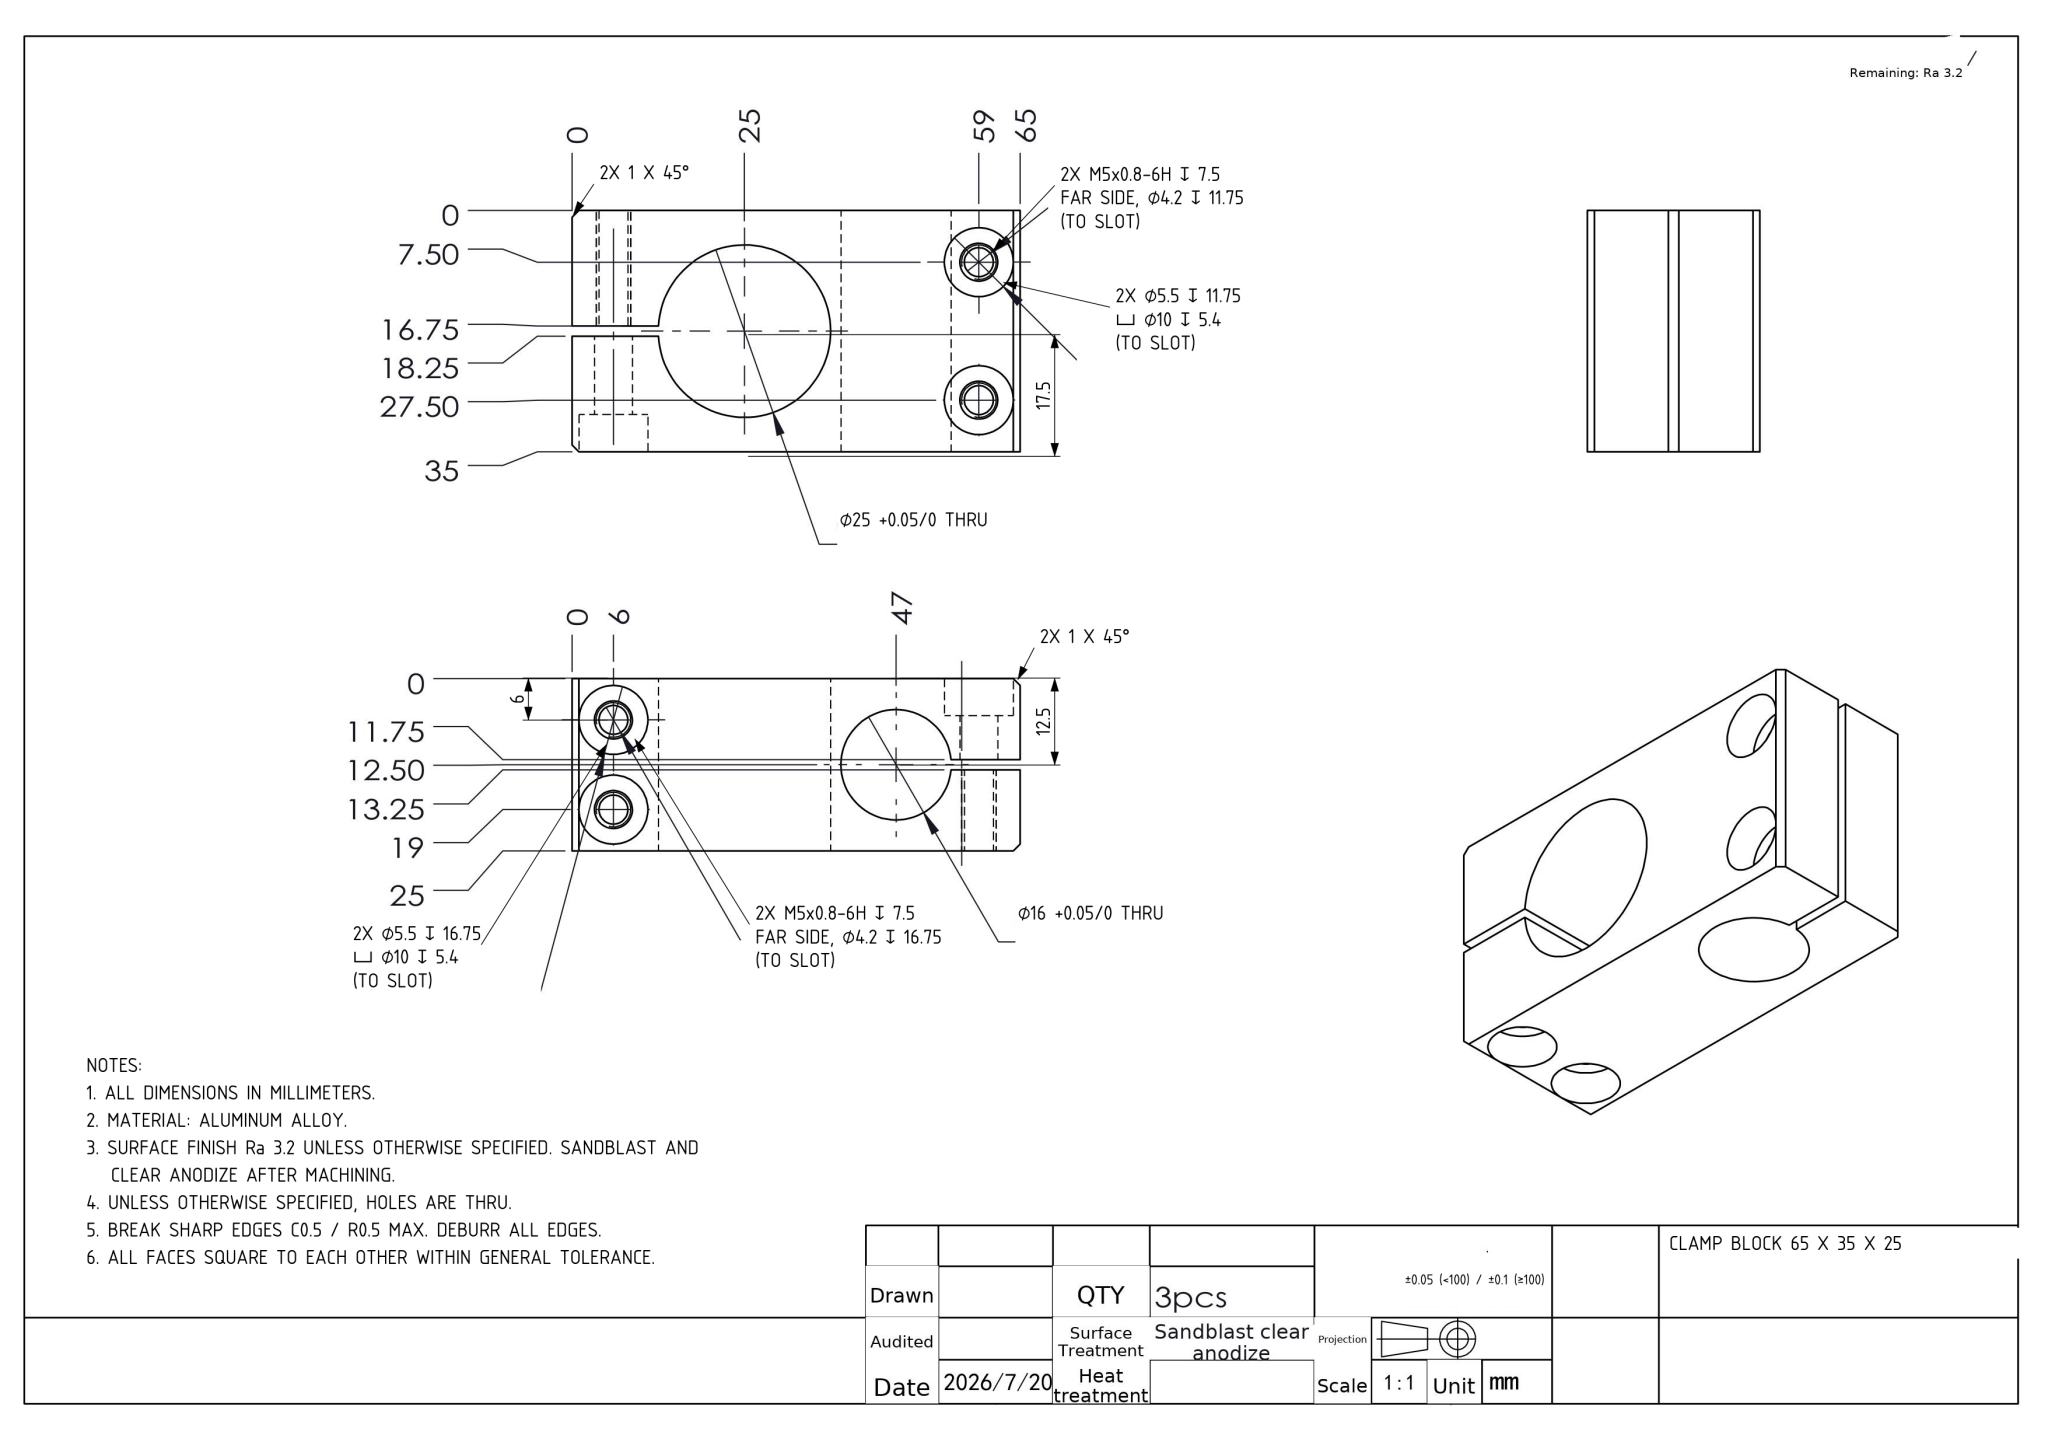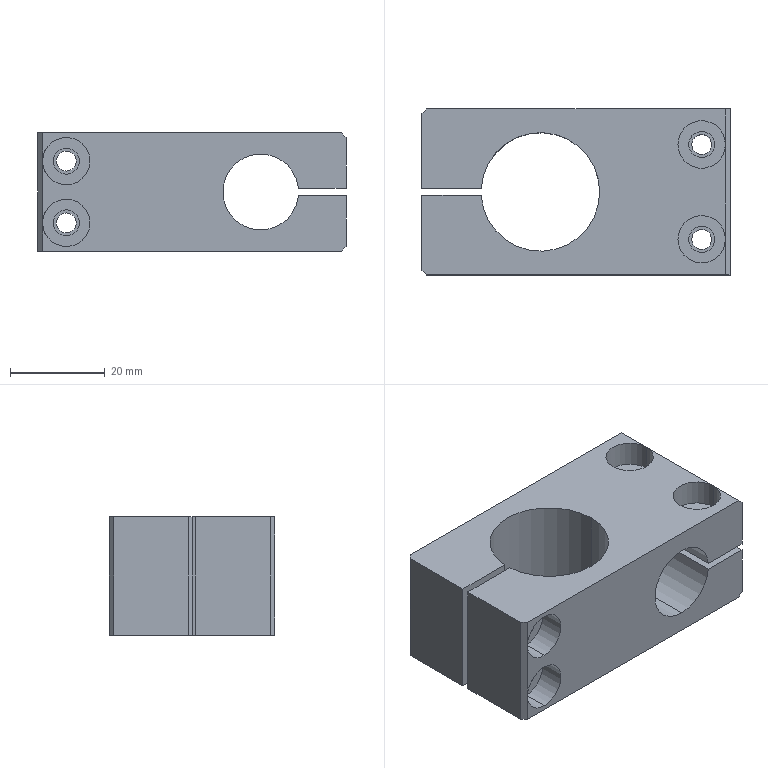Part | NX | mm | 1 solid | 49 faces | box 65 x 35 x 25 mm | volume 33184 mm3 | cylinder 29 | plane 20 | commonest cylinder face diameters 4.2 x8 10 x8 5.5 x8 16 x3 25 x2